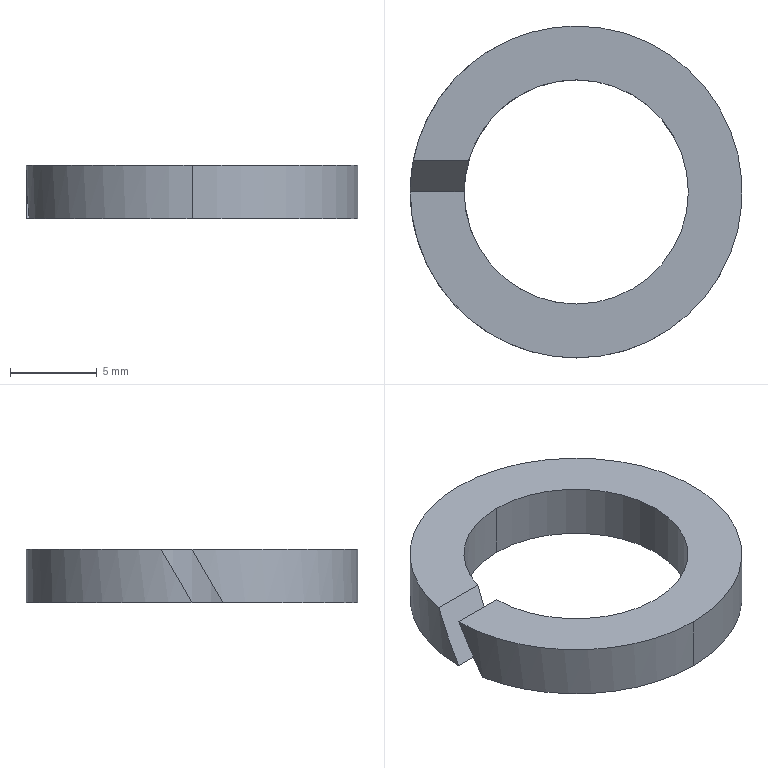Component | SolidWorks | Cylinder-1_spring lock washers--normal type gb-1 | 1 solid | 10 faces | box 19.1 x 19.1 x 3.1 mm | volume 466 mm3 | cylinder 6 | plane 4 | commonest cylinder face diameters 12.9 x3 19.1 x3
STEP:
#1=CARTESIAN_POINT('',(-8.211,0.1914,-6.86));
#2=VERTEX_POINT('',#1);
#3=CARTESIAN_POINT('',(-8.211,-0.3165,-6.86));
#4=VERTEX_POINT('',#3);
#5=CARTESIAN_POINT('',(-8.211,-0.06252,-6.86));
#6=DIRECTION('',(-0.,-0.,-1.));
#7=DIRECTION('',(0.,-1.,0.));
#8=AXIS2_PLACEMENT_3D('',#5,#6,#7);
#9=CIRCLE('',#8,0.2539);
#10=EDGE_CURVE('',#2,#4,#9,.T.);
#11=ORIENTED_EDGE('',*,*,#10,.F.);
#12=CARTESIAN_POINT('',(-8.211,0.1914,-6.982));
#13=VERTEX_POINT('',#12);
#14=CARTESIAN_POINT('',(-8.211,0.1914,-6.86));
#15=DIRECTION('',(-0.,-0.,-1.));
#16=VECTOR('',#15,39.37);
#17=LINE('',#14,#16);
#18=EDGE_CURVE('',#2,#13,#17,.T.);
#19=ORIENTED_EDGE('',*,*,#18,.T.);
#20=CARTESIAN_POINT('',(-8.211,-0.3165,-6.982));
#21=VERTEX_POINT('',#20);
#22=CARTESIAN_POINT('',(-8.211,-0.06252,-6.982));
#23=DIRECTION('',(-0.,-0.,-1.));
#24=DIRECTION('',(0.,-1.,0.));
#25=AXIS2_PLACEMENT_3D('',#22,#23,#24);
#26=CIRCLE('',#25,0.2539);
#27=EDGE_CURVE('',#13,#21,#26,.T.);
#28=ORIENTED_EDGE('',*,*,#27,.T.);
#29=CARTESIAN_POINT('',(-8.211,-0.3165,-6.86));
#30=DIRECTION('',(-0.,-0.,-1.));
#31=VECTOR('',#30,39.37);
#32=LINE('',#29,#31);
#33=EDGE_CURVE('',#4,#21,#32,.T.);
#34=ORIENTED_EDGE('',*,*,#33,.F.);
#35=EDGE_LOOP('',(#11,#19,#28,#34));
#36=FACE_OUTER_BOUND('',#35,.T.);
#37=CARTESIAN_POINT('',(-8.211,-0.06252,-6.86));
#38=DIRECTION('',(-0.,-0.,-1.));
#39=DIRECTION('',(0.,-1.,0.));
#40=AXIS2_PLACEMENT_3D('',#37,#38,#39);
#41=CYLINDRICAL_SURFACE('',#40,0.2539);
#42=ADVANCED_FACE('',(#36),#41,.F.);
#43=CARTESIAN_POINT('',(-8.465,-0.06252,-6.86));
#44=VERTEX_POINT('',#43);
#45=CARTESIAN_POINT('',(-8.211,-0.06252,-6.86));
#46=DIRECTION('',(-0.,-0.,-1.));
#47=DIRECTION('',(0.,-1.,0.));
#48=AXIS2_PLACEMENT_3D('',#45,#46,#47);
#49=CIRCLE('',#48,0.2539);
#50=EDGE_CURVE('',#4,#44,#49,.T.);
#51=ORIENTED_EDGE('',*,*,#50,.F.);
#52=ORIENTED_EDGE('',*,*,#33,.T.);
#53=CARTESIAN_POINT('',(-8.455,-0.133,-6.982));
#54=VERTEX_POINT('',#53);
#55=CARTESIAN_POINT('',(-8.211,-0.06252,-6.982));
#56=DIRECTION('',(-0.,-0.,-1.));
#57=DIRECTION('',(0.,-1.,0.));
#58=AXIS2_PLACEMENT_3D('',#55,#56,#57);
#59=CIRCLE('',#58,0.2539);
#60=EDGE_CURVE('',#21,#54,#59,.T.);
#61=ORIENTED_EDGE('',*,*,#60,.T.);
#62=CARTESIAN_POINT('',(-8.465,-0.06252,-6.86));
#63=CARTESIAN_POINT('',(-8.465,-0.0864,-6.902));
#64=CARTESIAN_POINT('',(-8.461,-0.11,-6.943));
#65=CARTESIAN_POINT('',(-8.455,-0.133,-6.982));
#66=(BOUNDED_CURVE()B_SPLINE_CURVE(3,(#62,#63,#64,#65),.UNSPECIFIED.,.F.,.F.)B_SPLINE_CURVE_WITH_KNOTS((4,4),(4.712,4.994),.UNSPECIFIED.)CURVE()GEOMETRIC_REPRESENTATION_ITEM()RATIONAL_B_SPLINE_CURVE((1.,0.9934,0.9934,1.))REPRESENTATION_ITEM(''));
#67=EDGE_CURVE('',#44,#54,#66,.T.);
#68=ORIENTED_EDGE('',*,*,#67,.F.);
#69=EDGE_LOOP('',(#51,#52,#61,#68));
#70=FACE_OUTER_BOUND('',#69,.T.);
#71=CARTESIAN_POINT('',(-8.211,-0.06252,-6.86));
#72=DIRECTION('',(-0.,-0.,-1.));
#73=DIRECTION('',(0.,-1.,0.));
#74=AXIS2_PLACEMENT_3D('',#71,#72,#73);
#75=CYLINDRICAL_SURFACE('',#74,0.2539);
#76=ADVANCED_FACE('',(#70),#75,.F.);
#77=CARTESIAN_POINT('',(-8.58,0.00794,-6.86));
#78=VERTEX_POINT('',#77);
#79=CARTESIAN_POINT('',(-8.211,0.3135,-6.86));
#80=VERTEX_POINT('',#79);
#81=CARTESIAN_POINT('',(-8.211,-0.06252,-6.86));
#82=DIRECTION('',(-0.,-0.,-1.));
#83=DIRECTION('',(0.,-1.,0.));
#84=AXIS2_PLACEMENT_3D('',#81,#82,#83);
#85=CIRCLE('',#84,0.376);
#86=EDGE_CURVE('',#78,#80,#85,.T.);
#87=ORIENTED_EDGE('',*,*,#86,.T.);
#88=CARTESIAN_POINT('',(-8.211,0.3135,-6.982));
#89=VERTEX_POINT('',#88);
#90=CARTESIAN_POINT('',(-8.211,0.3135,-6.86));
#91=DIRECTION('',(-0.,-0.,-1.));
#92=VECTOR('',#91,39.37);
#93=LINE('',#90,#92);
#94=EDGE_CURVE('',#80,#89,#93,.T.);
#95=ORIENTED_EDGE('',*,*,#94,.T.);
#96=CARTESIAN_POINT('',(-8.587,-0.06252,-6.982));
#97=VERTEX_POINT('',#96);
#98=CARTESIAN_POINT('',(-8.211,-0.06252,-6.982));
#99=DIRECTION('',(-0.,-0.,-1.));
#100=DIRECTION('',(0.,-1.,0.));
#101=AXIS2_PLACEMENT_3D('',#98,#99,#100);
#102=CIRCLE('',#101,0.376);
#103=EDGE_CURVE('',#97,#89,#102,.T.);
#104=ORIENTED_EDGE('',*,*,#103,.F.);
#105=CARTESIAN_POINT('',(-8.587,-0.06252,-6.982));
#106=CARTESIAN_POINT('',(-8.587,-0.03886,-6.941));
#107=CARTESIAN_POINT('',(-8.585,-0.0153,-6.901));
#108=CARTESIAN_POINT('',(-8.58,0.00794,-6.86));
#109=(BOUNDED_CURVE()B_SPLINE_CURVE(3,(#105,#106,#107,#108),.UNSPECIFIED.,.F.,.F.)B_SPLINE_CURVE_WITH_KNOTS((4,4),(1.571,1.759),.UNSPECIFIED.)CURVE()GEOMETRIC_REPRESENTATION_ITEM()RATIONAL_B_SPLINE_CURVE((1.,0.997,0.997,1.))REPRESENTATION_ITEM(''));
#110=EDGE_CURVE('',#97,#78,#109,.T.);
#111=ORIENTED_EDGE('',*,*,#110,.T.);
#112=EDGE_LOOP('',(#87,#95,#104,#111));
#113=FACE_OUTER_BOUND('',#112,.T.);
#114=CARTESIAN_POINT('',(-8.211,-0.06252,-6.86));
#115=DIRECTION('',(-0.,-0.,-1.));
#116=DIRECTION('',(0.,-1.,0.));
#117=AXIS2_PLACEMENT_3D('',#114,#115,#116);
#118=CYLINDRICAL_SURFACE('',#117,0.376);
#119=ADVANCED_FACE('',(#113),#118,.T.);
#120=ORIENTED_EDGE('',*,*,#94,.F.);
#121=CARTESIAN_POINT('',(-8.211,-0.4385,-6.86));
#122=VERTEX_POINT('',#121);
#123=CARTESIAN_POINT('',(-8.211,-0.06252,-6.86));
#124=DIRECTION('',(-0.,-0.,-1.));
#125=DIRECTION('',(0.,-1.,0.));
#126=AXIS2_PLACEMENT_3D('',#123,#124,#125);
#127=CIRCLE('',#126,0.376);
#128=EDGE_CURVE('',#80,#122,#127,.T.);
#129=ORIENTED_EDGE('',*,*,#128,.T.);
#130=CARTESIAN_POINT('',(-8.211,-0.4385,-6.982));
#131=VERTEX_POINT('',#130);
#132=CARTESIAN_POINT('',(-8.211,-0.4385,-6.86));
#133=DIRECTION('',(-0.,-0.,-1.));
#134=VECTOR('',#133,39.37);
#135=LINE('',#132,#134);
#136=EDGE_CURVE('',#122,#131,#135,.T.);
#137=ORIENTED_EDGE('',*,*,#136,.T.);
#138=CARTESIAN_POINT('',(-8.211,-0.06252,-6.982));
#139=DIRECTION('',(-0.,-0.,-1.));
#140=DIRECTION('',(0.,-1.,0.));
#141=AXIS2_PLACEMENT_3D('',#138,#139,#140);
#142=CIRCLE('',#141,0.376);
#143=EDGE_CURVE('',#89,#131,#142,.T.);
#144=ORIENTED_EDGE('',*,*,#143,.F.);
#145=EDGE_LOOP('',(#120,#129,#137,#144));
#146=FACE_OUTER_BOUND('',#145,.T.);
#147=CARTESIAN_POINT('',(-8.211,-0.06252,-6.86));
#148=DIRECTION('',(-0.,-0.,-1.));
#149=DIRECTION('',(0.,-1.,0.));
#150=AXIS2_PLACEMENT_3D('',#147,#148,#149);
#151=CYLINDRICAL_SURFACE('',#150,0.376);
#152=ADVANCED_FACE('',(#146),#151,.T.);
#153=ORIENTED_EDGE('',*,*,#136,.F.);
#154=CARTESIAN_POINT('',(-8.587,-0.06252,-6.86));
#155=VERTEX_POINT('',#154);
#156=CARTESIAN_POINT('',(-8.211,-0.06252,-6.86));
#157=DIRECTION('',(-0.,-0.,-1.));
#158=DIRECTION('',(0.,-1.,0.));
#159=AXIS2_PLACEMENT_3D('',#156,#157,#158);
#160=CIRCLE('',#159,0.376);
#161=EDGE_CURVE('',#122,#155,#160,.T.);
#162=ORIENTED_EDGE('',*,*,#161,.T.);
#163=CARTESIAN_POINT('',(-8.58,-0.133,-6.982));
#164=VERTEX_POINT('',#163);
#165=CARTESIAN_POINT('',(-8.587,-0.06252,-6.86));
#166=CARTESIAN_POINT('',(-8.587,-0.08619,-6.901));
#167=CARTESIAN_POINT('',(-8.585,-0.1097,-6.942));
#168=CARTESIAN_POINT('',(-8.58,-0.133,-6.982));
#169=(BOUNDED_CURVE()B_SPLINE_CURVE(3,(#165,#166,#167,#168),.UNSPECIFIED.,.F.,.F.)B_SPLINE_CURVE_WITH_KNOTS((4,4),(4.712,4.901),.UNSPECIFIED.)CURVE()GEOMETRIC_REPRESENTATION_ITEM()RATIONAL_B_SPLINE_CURVE((1.,0.997,0.997,1.))REPRESENTATION_ITEM(''));
#170=EDGE_CURVE('',#155,#164,#169,.T.);
#171=ORIENTED_EDGE('',*,*,#170,.T.);
#172=CARTESIAN_POINT('',(-8.211,-0.06252,-6.982));
#173=DIRECTION('',(-0.,-0.,-1.));
#174=DIRECTION('',(0.,-1.,0.));
#175=AXIS2_PLACEMENT_3D('',#172,#173,#174);
#176=CIRCLE('',#175,0.376);
#177=EDGE_CURVE('',#131,#164,#176,.T.);
#178=ORIENTED_EDGE('',*,*,#177,.F.);
#179=EDGE_LOOP('',(#153,#162,#171,#178));
#180=FACE_OUTER_BOUND('',#179,.T.);
#181=CARTESIAN_POINT('',(-8.211,-0.06252,-6.86));
#182=DIRECTION('',(-0.,-0.,-1.));
#183=DIRECTION('',(0.,-1.,0.));
#184=AXIS2_PLACEMENT_3D('',#181,#182,#183);
#185=CYLINDRICAL_SURFACE('',#184,0.376);
#186=ADVANCED_FACE('',(#180),#185,.T.);
#187=CARTESIAN_POINT('',(-8.455,0.00794,-6.86));
#188=VERTEX_POINT('',#187);
#189=CARTESIAN_POINT('',(-8.587,0.00794,-6.86));
#190=DIRECTION('',(1.,0.,-0.));
#191=VECTOR('',#190,39.37);
#192=LINE('',#189,#191);
#193=EDGE_CURVE('',#78,#188,#192,.T.);
#194=ORIENTED_EDGE('',*,*,#193,.T.);
#195=CARTESIAN_POINT('',(-8.211,-0.06252,-6.86));
#196=DIRECTION('',(-0.,-0.,-1.));
#197=DIRECTION('',(0.,-1.,0.));
#198=AXIS2_PLACEMENT_3D('',#195,#196,#197);
#199=CIRCLE('',#198,0.2539);
#200=EDGE_CURVE('',#188,#2,#199,.T.);
#201=ORIENTED_EDGE('',*,*,#200,.T.);
#202=ORIENTED_EDGE('',*,*,#10,.T.);
#203=ORIENTED_EDGE('',*,*,#50,.T.);
#204=CARTESIAN_POINT('',(-8.587,-0.06252,-6.86));
#205=DIRECTION('',(1.,0.,-0.));
#206=VECTOR('',#205,39.37);
#207=LINE('',#204,#206);
#208=EDGE_CURVE('',#155,#44,#207,.T.);
#209=ORIENTED_EDGE('',*,*,#208,.F.);
#210=ORIENTED_EDGE('',*,*,#161,.F.);
#211=ORIENTED_EDGE('',*,*,#128,.F.);
#212=ORIENTED_EDGE('',*,*,#86,.F.);
#213=EDGE_LOOP('',(#194,#201,#202,#203,#209,#210,#211,#212));
#214=FACE_OUTER_BOUND('',#213,.T.);
#215=CARTESIAN_POINT('',(-8.211,-0.06252,-6.86));
#216=DIRECTION('',(-0.,-0.,-1.));
#217=DIRECTION('',(0.,-1.,0.));
#218=AXIS2_PLACEMENT_3D('',#215,#216,#217);
#219=PLANE('',#218);
#220=ADVANCED_FACE('',(#214),#219,.F.);
#221=CARTESIAN_POINT('',(-8.465,-0.06252,-6.982));
#222=VERTEX_POINT('',#221);
#223=CARTESIAN_POINT('',(-8.211,-0.06252,-6.982));
#224=DIRECTION('',(-0.,-0.,-1.));
#225=DIRECTION('',(0.,-1.,0.));
#226=AXIS2_PLACEMENT_3D('',#223,#224,#225);
#227=CIRCLE('',#226,0.2539);
#228=EDGE_CURVE('',#222,#13,#227,.T.);
#229=ORIENTED_EDGE('',*,*,#228,.F.);
#230=CARTESIAN_POINT('',(-8.587,-0.06252,-6.982));
#231=DIRECTION('',(1.,0.,-0.));
#232=VECTOR('',#231,39.37);
#233=LINE('',#230,#232);
#234=EDGE_CURVE('',#97,#222,#233,.T.);
#235=ORIENTED_EDGE('',*,*,#234,.F.);
#236=ORIENTED_EDGE('',*,*,#103,.T.);
#237=ORIENTED_EDGE('',*,*,#143,.T.);
#238=ORIENTED_EDGE('',*,*,#177,.T.);
#239=CARTESIAN_POINT('',(-8.587,-0.133,-6.982));
#240=DIRECTION('',(1.,0.,-0.));
#241=VECTOR('',#240,39.37);
#242=LINE('',#239,#241);
#243=EDGE_CURVE('',#164,#54,#242,.T.);
#244=ORIENTED_EDGE('',*,*,#243,.T.);
#245=ORIENTED_EDGE('',*,*,#60,.F.);
#246=ORIENTED_EDGE('',*,*,#27,.F.);
#247=EDGE_LOOP('',(#229,#235,#236,#237,#238,#244,#245,#246));
#248=FACE_OUTER_BOUND('',#247,.T.);
#249=CARTESIAN_POINT('',(-8.211,-0.06252,-6.982));
#250=DIRECTION('',(-0.,-0.,-1.));
#251=DIRECTION('',(0.,-1.,0.));
#252=AXIS2_PLACEMENT_3D('',#249,#250,#251);
#253=PLANE('',#252);
#254=ADVANCED_FACE('',(#248),#253,.T.);
#255=ORIENTED_EDGE('',*,*,#18,.F.);
#256=ORIENTED_EDGE('',*,*,#200,.F.);
#257=CARTESIAN_POINT('',(-8.465,-0.06252,-6.982));
#258=CARTESIAN_POINT('',(-8.465,-0.03864,-6.941));
#259=CARTESIAN_POINT('',(-8.461,-0.015,-6.9));
#260=CARTESIAN_POINT('',(-8.455,0.00794,-6.86));
#261=(BOUNDED_CURVE()B_SPLINE_CURVE(3,(#257,#258,#259,#260),.UNSPECIFIED.,.F.,.F.)B_SPLINE_CURVE_WITH_KNOTS((4,4),(1.571,1.852),.UNSPECIFIED.)CURVE()GEOMETRIC_REPRESENTATION_ITEM()RATIONAL_B_SPLINE_CURVE((1.,0.9934,0.9934,1.))REPRESENTATION_ITEM(''));
#262=EDGE_CURVE('',#222,#188,#261,.T.);
#263=ORIENTED_EDGE('',*,*,#262,.F.);
#264=ORIENTED_EDGE('',*,*,#228,.T.);
#265=EDGE_LOOP('',(#255,#256,#263,#264));
#266=FACE_OUTER_BOUND('',#265,.T.);
#267=CARTESIAN_POINT('',(-8.211,-0.06252,-6.86));
#268=DIRECTION('',(-0.,-0.,-1.));
#269=DIRECTION('',(0.,-1.,0.));
#270=AXIS2_PLACEMENT_3D('',#267,#268,#269);
#271=CYLINDRICAL_SURFACE('',#270,0.2539);
#272=ADVANCED_FACE('',(#266),#271,.F.);
#273=ORIENTED_EDGE('',*,*,#208,.T.);
#274=ORIENTED_EDGE('',*,*,#67,.T.);
#275=ORIENTED_EDGE('',*,*,#243,.F.);
#276=ORIENTED_EDGE('',*,*,#170,.F.);
#277=EDGE_LOOP('',(#273,#274,#275,#276));
#278=FACE_OUTER_BOUND('',#277,.T.);
#279=CARTESIAN_POINT('',(-8.587,-0.06252,-6.86));
#280=DIRECTION('',(-0.,0.866,-0.5));
#281=DIRECTION('',(-0.,-0.5,-0.866));
#282=AXIS2_PLACEMENT_3D('',#279,#280,#281);
#283=PLANE('',#282);
#284=ADVANCED_FACE('',(#278),#283,.T.);
#285=ORIENTED_EDGE('',*,*,#234,.T.);
#286=ORIENTED_EDGE('',*,*,#262,.T.);
#287=ORIENTED_EDGE('',*,*,#193,.F.);
#288=ORIENTED_EDGE('',*,*,#110,.F.);
#289=EDGE_LOOP('',(#285,#286,#287,#288));
#290=FACE_OUTER_BOUND('',#289,.T.);
#291=CARTESIAN_POINT('',(-8.587,-0.06252,-6.982));
#292=DIRECTION('',(0.,-0.866,0.5));
#293=DIRECTION('',(0.,0.5,0.866));
#294=AXIS2_PLACEMENT_3D('',#291,#292,#293);
#295=PLANE('',#294);
#296=ADVANCED_FACE('',(#290),#295,.T.);
#297=CLOSED_SHELL('',(#42,#76,#119,#152,#186,#220,#254,#272,#284,#296));
#298=MANIFOLD_SOLID_BREP('',#297);
#299=CARTESIAN_POINT('',(0.,0.,0.));
#300=DIRECTION('',(0.,0.,1.));
#301=DIRECTION('',(1.,0.,0.));
#302=AXIS2_PLACEMENT_3D('',#299,#300,#301);
#303=(LENGTH_UNIT()NAMED_UNIT(*)SI_UNIT($,.METRE.));
#304=LENGTH_MEASURE_WITH_UNIT(LENGTH_MEASURE(0.0254),#303);
#305=DIMENSIONAL_EXPONENTS(1.,0.,0.,0.,0.,0.,0.);
#306=(CONVERSION_BASED_UNIT('',#304)LENGTH_UNIT()NAMED_UNIT(#305));
#307=UNCERTAINTY_MEASURE_WITH_UNIT(LENGTH_MEASURE(0.00001),#306,'','');
#308=(NAMED_UNIT(*)PLANE_ANGLE_UNIT()SI_UNIT($,.RADIAN.));
#309=(NAMED_UNIT(*)SI_UNIT($,.STERADIAN.)SOLID_ANGLE_UNIT());
#310=(GEOMETRIC_REPRESENTATION_CONTEXT(3)GLOBAL_UNCERTAINTY_ASSIGNED_CONTEXT((#307))GLOBAL_UNIT_ASSIGNED_CONTEXT((#306,#308,#309))REPRESENTATION_CONTEXT('',''));
#311=ADVANCED_BREP_SHAPE_REPRESENTATION('',(#298,#302),#310);
#312=COLOUR_RGB('',0.7922,0.8196,0.9333);
#313=FILL_AREA_STYLE_COLOUR('',#312);
#314=FILL_AREA_STYLE('',(#313));
#315=SURFACE_STYLE_FILL_AREA(#314);
#316=SURFACE_SIDE_STYLE('',(#315));
#317=SURFACE_STYLE_USAGE(.BOTH.,#316);
#318=PRESENTATION_STYLE_ASSIGNMENT((#317));
#319=STYLED_ITEM('',(#318),#298);
#320=PRESENTATION_LAYER_ASSIGNMENT('','',(#319));
#321=(LENGTH_UNIT()NAMED_UNIT(*)SI_UNIT($,.METRE.));
#322=LENGTH_MEASURE_WITH_UNIT(LENGTH_MEASURE(0.0254),#321);
#323=DIMENSIONAL_EXPONENTS(1.,0.,0.,0.,0.,0.,0.);
#324=(CONVERSION_BASED_UNIT('',#322)LENGTH_UNIT()NAMED_UNIT(#323));
#325=UNCERTAINTY_MEASURE_WITH_UNIT(LENGTH_MEASURE(0.00001),#324,'','');
#326=(NAMED_UNIT(*)PLANE_ANGLE_UNIT()SI_UNIT($,.RADIAN.));
#327=(NAMED_UNIT(*)SI_UNIT($,.STERADIAN.)SOLID_ANGLE_UNIT());
#328=(GEOMETRIC_REPRESENTATION_CONTEXT(3)GLOBAL_UNCERTAINTY_ASSIGNED_CONTEXT((#325))GLOBAL_UNIT_ASSIGNED_CONTEXT((#324,#326,#327))REPRESENTATION_CONTEXT('',''));
#329=MECHANICAL_DESIGN_GEOMETRIC_PRESENTATION_REPRESENTATION('',(#319),#328);